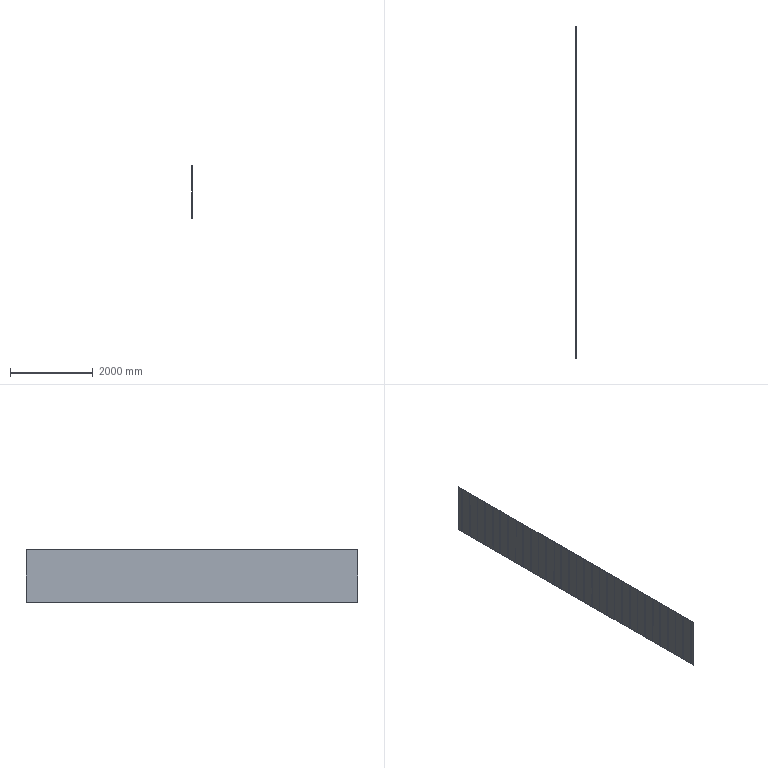Component | SolidWorks | 8mTread-3 | 1 solid | 130 faces | box 8 x 8009.05 x 1257 mm | volume 78214286 mm3 | plane 130
build123d program:
from build123d import *

# Parameters (mm, degrees)
BOSS_EXTRUDE1_DEPTH     = 8
SKETCH2_W               = 1638.54
SKETCH2_H               = 30
CUT_EXTRUDE_THIN1_DEPTH = 2
LPATTERN1_COUNT         = 31
LPATTERN1_PITCH         = 260


with BuildPart() as part:
    # Sketch1 → Boss-Extrude1 (new body)
    with BuildSketch(Plane.XY):
        Polygon((-4933.447, 9723.056), (-6190.447, 9723.056), (-6190.447, 15723.056), (-6190.447, 17732.107), (-4933.447, 17732.107), (-4933.447, 14990.845), align=None)
    extrude(amount=BOSS_EXTRUDE1_DEPTH)

    # Sketch2 → Cut-Extrude-Thin1 (cut)
    with BuildSketch(Plane(origin=(0, 0, 0), x_dir=(-1, 0, 0), z_dir=(0, 0, -1))):
        with Locations((5364.03, 9846.058)):
            Rectangle(SKETCH2_W, SKETCH2_H)
    cut_extrude_thin1 = extrude(amount=-CUT_EXTRUDE_THIN1_DEPTH, mode=Mode.SUBTRACT)

    # LPattern1: Cut-Extrude-Thin1 ×31
    with Locations(*[(0, i * LPATTERN1_PITCH, 0) for i in range(1, LPATTERN1_COUNT)]):
        add(cut_extrude_thin1, mode=Mode.SUBTRACT)


solid = part.part

# Placed as in the assembly
solid = solid.moved(Location((2077.926, -13426.79, -2234.447), (180, -90, 0)))